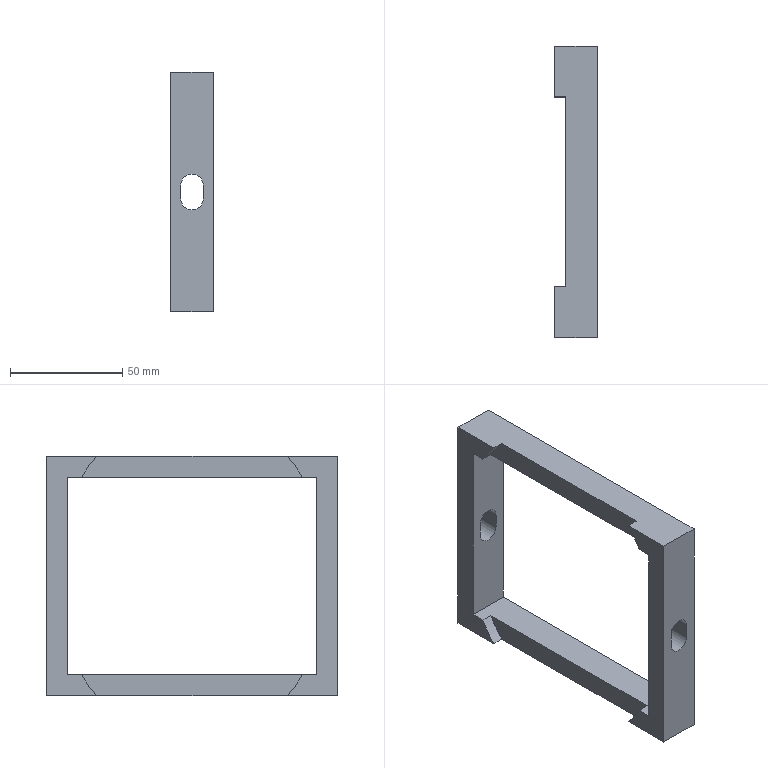Component | NX | FRAME | 1 solid | 25 faces | volume 67293 mm3 | plane 17 | cylinder 8 | commonest cylinder face diameters 114 x4 10 x4